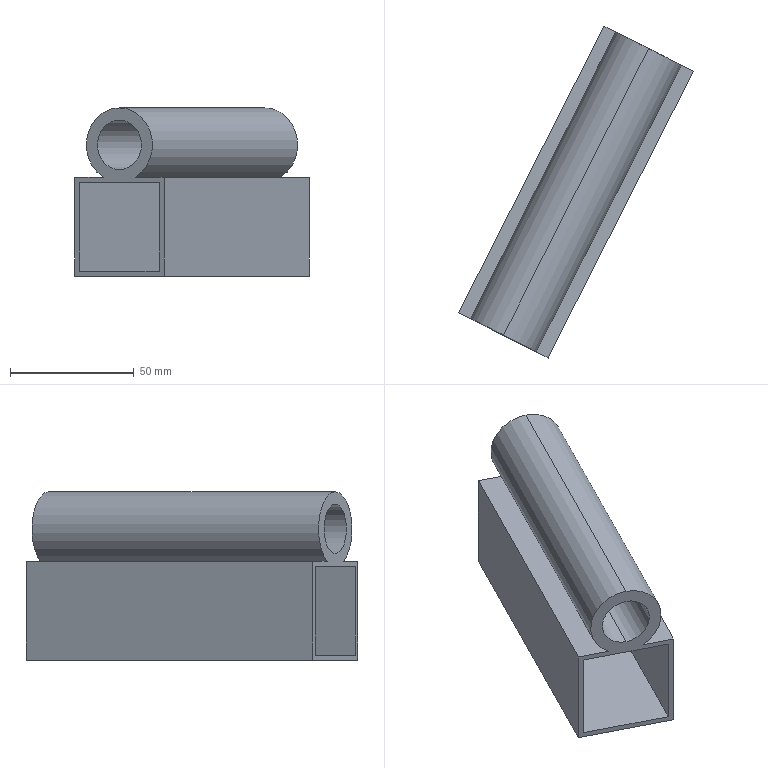Component | SolidWorks | Assembly4-1_Part24-1 | 1 solid | 15 faces | box 94.94 x 134.29 x 68.11 mm | volume 90975 mm3 | plane 11 | cylinder 4 | commonest cylinder face diameters 20 x2 30 x2
build123d program:
from build123d import *

# Parameters (mm, degrees)
SKETCH3_R           = 10
SKETCH3_W           = 36
SKETCH3_H           = 36
BOSS_EXTRUDE5_DEPTH = 130


with BuildPart() as part:
    # Sketch3 → Boss-Extrude5 (new body)
    with BuildSketch(Plane.XY):
        with BuildLine():
            Line((-59.292, 37.231), (-19.292, 37.231))
            Line((-19.292, 37.231), (-19.292, -3.313))
            Line((-19.292, -3.313), (-59.292, -3.313))
            Line((-59.292, -3.313), (-59.292, 9.667))
            ThreePointArc((-59.292, 9.667), (-87.4, 16.959), (-59.292, 24.251))
            Line((-59.292, 24.251), (-59.292, 37.231))
        make_face()
        with Locations((-72.4, 16.959)):
            Circle(SKETCH3_R, mode=Mode.SUBTRACT)
        with Locations((-39.292, 16.959)):
            Rectangle(SKETCH3_W, SKETCH3_H, mode=Mode.SUBTRACT)
    extrude(amount=BOSS_EXTRUDE5_DEPTH)


solid = part.part

# Placed as in the assembly
solid = solid.moved(Location((-428.429, -861.036, 1016.679), (90, -26.879, -90)))
STEP:
#1=CARTESIAN_POINT('',(-18.586,-38.766,43.271));
#2=VERTEX_POINT('',#1);
#3=CARTESIAN_POINT('',(-18.586,-38.766,42.483));
#4=VERTEX_POINT('',#3);
#5=CARTESIAN_POINT('',(-18.586,-38.766,42.877));
#6=DIRECTION('',(-0.4521,-0.892,-0.));
#7=DIRECTION('',(0.,0.,-1.));
#8=AXIS2_PLACEMENT_3D('',#5,#6,#7);
#9=CIRCLE('',#8,0.3937);
#10=EDGE_CURVE('',#2,#4,#9,.T.);
#11=ORIENTED_EDGE('',*,*,#10,.T.);
#12=CARTESIAN_POINT('',(-16.272,-34.201,42.483));
#13=VERTEX_POINT('',#12);
#14=CARTESIAN_POINT('',(-18.586,-38.766,42.483));
#15=DIRECTION('',(0.4521,0.892,0.));
#16=VECTOR('',#15,39.37);
#17=LINE('',#14,#16);
#18=EDGE_CURVE('',#4,#13,#17,.T.);
#19=ORIENTED_EDGE('',*,*,#18,.T.);
#20=CARTESIAN_POINT('',(-16.272,-34.201,43.271));
#21=VERTEX_POINT('',#20);
#22=CARTESIAN_POINT('',(-16.272,-34.201,42.877));
#23=DIRECTION('',(-0.4521,-0.892,-0.));
#24=DIRECTION('',(0.,0.,-1.));
#25=AXIS2_PLACEMENT_3D('',#22,#23,#24);
#26=CIRCLE('',#25,0.3937);
#27=EDGE_CURVE('',#21,#13,#26,.T.);
#28=ORIENTED_EDGE('',*,*,#27,.F.);
#29=CARTESIAN_POINT('',(-18.586,-38.766,43.271));
#30=DIRECTION('',(0.4521,0.892,0.));
#31=VECTOR('',#30,39.37);
#32=LINE('',#29,#31);
#33=EDGE_CURVE('',#2,#21,#32,.T.);
#34=ORIENTED_EDGE('',*,*,#33,.F.);
#35=EDGE_LOOP('',(#11,#19,#28,#34));
#36=FACE_OUTER_BOUND('',#35,.T.);
#37=CARTESIAN_POINT('',(-18.586,-38.766,42.877));
#38=DIRECTION('',(0.4521,0.892,0.));
#39=DIRECTION('',(-0.,-0.,1.));
#40=AXIS2_PLACEMENT_3D('',#37,#38,#39);
#41=CYLINDRICAL_SURFACE('',#40,0.3937);
#42=ADVANCED_FACE('',(#36),#41,.F.);
#43=CARTESIAN_POINT('',(-18.586,-38.766,43.468));
#44=VERTEX_POINT('',#43);
#45=CARTESIAN_POINT('',(-18.842,-38.636,42.361));
#46=VERTEX_POINT('',#45);
#47=CARTESIAN_POINT('',(-18.586,-38.766,42.877));
#48=DIRECTION('',(-0.4521,-0.892,-0.));
#49=DIRECTION('',(0.,0.,-1.));
#50=AXIS2_PLACEMENT_3D('',#47,#48,#49);
#51=CIRCLE('',#50,0.5906);
#52=EDGE_CURVE('',#44,#46,#51,.T.);
#53=ORIENTED_EDGE('',*,*,#52,.F.);
#54=CARTESIAN_POINT('',(-16.272,-34.201,43.468));
#55=VERTEX_POINT('',#54);
#56=CARTESIAN_POINT('',(-18.586,-38.766,43.468));
#57=DIRECTION('',(0.4521,0.892,0.));
#58=VECTOR('',#57,39.37);
#59=LINE('',#56,#58);
#60=EDGE_CURVE('',#44,#55,#59,.T.);
#61=ORIENTED_EDGE('',*,*,#60,.T.);
#62=CARTESIAN_POINT('',(-16.528,-34.071,42.361));
#63=VERTEX_POINT('',#62);
#64=CARTESIAN_POINT('',(-16.272,-34.201,42.877));
#65=DIRECTION('',(-0.4521,-0.892,-0.));
#66=DIRECTION('',(0.,0.,-1.));
#67=AXIS2_PLACEMENT_3D('',#64,#65,#66);
#68=CIRCLE('',#67,0.5906);
#69=EDGE_CURVE('',#55,#63,#68,.T.);
#70=ORIENTED_EDGE('',*,*,#69,.T.);
#71=CARTESIAN_POINT('',(-18.842,-38.636,42.361));
#72=DIRECTION('',(0.4521,0.892,0.));
#73=VECTOR('',#72,39.37);
#74=LINE('',#71,#73);
#75=EDGE_CURVE('',#46,#63,#74,.T.);
#76=ORIENTED_EDGE('',*,*,#75,.F.);
#77=EDGE_LOOP('',(#53,#61,#70,#76));
#78=FACE_OUTER_BOUND('',#77,.T.);
#79=CARTESIAN_POINT('',(-18.586,-38.766,42.877));
#80=DIRECTION('',(0.4521,0.892,0.));
#81=DIRECTION('',(-0.,-0.,1.));
#82=AXIS2_PLACEMENT_3D('',#79,#80,#81);
#83=CYLINDRICAL_SURFACE('',#82,0.5906);
#84=ADVANCED_FACE('',(#78),#83,.T.);
#85=CARTESIAN_POINT('',(-17.874,-39.127,42.361));
#86=VERTEX_POINT('',#85);
#87=CARTESIAN_POINT('',(-18.33,-38.896,42.361));
#88=VERTEX_POINT('',#87);
#89=CARTESIAN_POINT('',(-17.874,-39.127,42.361));
#90=DIRECTION('',(-0.892,0.4521,0.));
#91=VECTOR('',#90,39.37);
#92=LINE('',#89,#91);
#93=EDGE_CURVE('',#86,#88,#92,.T.);
#94=ORIENTED_EDGE('',*,*,#93,.T.);
#95=CARTESIAN_POINT('',(-18.586,-38.766,42.877));
#96=DIRECTION('',(-0.4521,-0.892,-0.));
#97=DIRECTION('',(0.,0.,-1.));
#98=AXIS2_PLACEMENT_3D('',#95,#96,#97);
#99=CIRCLE('',#98,0.5906);
#100=EDGE_CURVE('',#88,#44,#99,.T.);
#101=ORIENTED_EDGE('',*,*,#100,.T.);
#102=ORIENTED_EDGE('',*,*,#52,.T.);
#103=CARTESIAN_POINT('',(-19.297,-38.405,42.361));
#104=VERTEX_POINT('',#103);
#105=CARTESIAN_POINT('',(-18.842,-38.636,42.361));
#106=DIRECTION('',(-0.892,0.4521,0.));
#107=VECTOR('',#106,39.37);
#108=LINE('',#105,#107);
#109=EDGE_CURVE('',#46,#104,#108,.T.);
#110=ORIENTED_EDGE('',*,*,#109,.T.);
#111=CARTESIAN_POINT('',(-19.297,-38.405,40.786));
#112=VERTEX_POINT('',#111);
#113=CARTESIAN_POINT('',(-19.297,-38.405,42.361));
#114=DIRECTION('',(0.,0.,-1.));
#115=VECTOR('',#114,39.37);
#116=LINE('',#113,#115);
#117=EDGE_CURVE('',#104,#112,#116,.T.);
#118=ORIENTED_EDGE('',*,*,#117,.T.);
#119=CARTESIAN_POINT('',(-17.874,-39.127,40.786));
#120=VERTEX_POINT('',#119);
#121=CARTESIAN_POINT('',(-17.874,-39.127,40.786));
#122=DIRECTION('',(0.892,-0.4521,-0.));
#123=VECTOR('',#122,39.37);
#124=LINE('',#121,#123);
#125=EDGE_CURVE('',#112,#120,#124,.T.);
#126=ORIENTED_EDGE('',*,*,#125,.T.);
#127=CARTESIAN_POINT('',(-17.874,-39.127,42.361));
#128=DIRECTION('',(-0.,-0.,1.));
#129=VECTOR('',#128,39.37);
#130=LINE('',#127,#129);
#131=EDGE_CURVE('',#120,#86,#130,.T.);
#132=ORIENTED_EDGE('',*,*,#131,.T.);
#133=EDGE_LOOP('',(#94,#101,#102,#110,#118,#126,#132));
#134=FACE_OUTER_BOUND('',#133,.T.);
#135=ORIENTED_EDGE('',*,*,#10,.F.);
#136=CARTESIAN_POINT('',(-18.586,-38.766,42.877));
#137=DIRECTION('',(-0.4521,-0.892,-0.));
#138=DIRECTION('',(0.,0.,-1.));
#139=AXIS2_PLACEMENT_3D('',#136,#137,#138);
#140=CIRCLE('',#139,0.3937);
#141=EDGE_CURVE('',#4,#2,#140,.T.);
#142=ORIENTED_EDGE('',*,*,#141,.F.);
#143=EDGE_LOOP('',(#135,#142));
#144=FACE_BOUND('',#143,.T.);
#145=CARTESIAN_POINT('',(-17.954,-39.086,40.865));
#146=VERTEX_POINT('',#145);
#147=CARTESIAN_POINT('',(-17.954,-39.086,42.282));
#148=VERTEX_POINT('',#147);
#149=CARTESIAN_POINT('',(-17.954,-39.086,42.282));
#150=DIRECTION('',(-0.,-0.,1.));
#151=VECTOR('',#150,39.37);
#152=LINE('',#149,#151);
#153=EDGE_CURVE('',#146,#148,#152,.T.);
#154=ORIENTED_EDGE('',*,*,#153,.F.);
#155=CARTESIAN_POINT('',(-19.218,-38.446,40.865));
#156=VERTEX_POINT('',#155);
#157=CARTESIAN_POINT('',(-17.954,-39.086,40.865));
#158=DIRECTION('',(0.892,-0.4521,-0.));
#159=VECTOR('',#158,39.37);
#160=LINE('',#157,#159);
#161=EDGE_CURVE('',#156,#146,#160,.T.);
#162=ORIENTED_EDGE('',*,*,#161,.F.);
#163=CARTESIAN_POINT('',(-19.218,-38.446,42.282));
#164=VERTEX_POINT('',#163);
#165=CARTESIAN_POINT('',(-19.218,-38.446,42.282));
#166=DIRECTION('',(0.,0.,-1.));
#167=VECTOR('',#166,39.37);
#168=LINE('',#165,#167);
#169=EDGE_CURVE('',#164,#156,#168,.T.);
#170=ORIENTED_EDGE('',*,*,#169,.F.);
#171=CARTESIAN_POINT('',(-17.954,-39.086,42.282));
#172=DIRECTION('',(-0.892,0.4521,0.));
#173=VECTOR('',#172,39.37);
#174=LINE('',#171,#173);
#175=EDGE_CURVE('',#148,#164,#174,.T.);
#176=ORIENTED_EDGE('',*,*,#175,.F.);
#177=EDGE_LOOP('',(#154,#162,#170,#176));
#178=FACE_BOUND('',#177,.T.);
#179=CARTESIAN_POINT('',(-18.586,-38.766,42.877));
#180=DIRECTION('',(-0.4521,-0.892,-0.));
#181=DIRECTION('',(0.,0.,-1.));
#182=AXIS2_PLACEMENT_3D('',#179,#180,#181);
#183=PLANE('',#182);
#184=ADVANCED_FACE('',(#134,#144,#178),#183,.T.);
#185=ORIENTED_EDGE('',*,*,#27,.T.);
#186=CARTESIAN_POINT('',(-16.272,-34.201,42.877));
#187=DIRECTION('',(-0.4521,-0.892,-0.));
#188=DIRECTION('',(0.,0.,-1.));
#189=AXIS2_PLACEMENT_3D('',#186,#187,#188);
#190=CIRCLE('',#189,0.3937);
#191=EDGE_CURVE('',#13,#21,#190,.T.);
#192=ORIENTED_EDGE('',*,*,#191,.T.);
#193=EDGE_LOOP('',(#185,#192));
#194=FACE_BOUND('',#193,.T.);
#195=CARTESIAN_POINT('',(-15.56,-34.562,42.361));
#196=VERTEX_POINT('',#195);
#197=CARTESIAN_POINT('',(-16.016,-34.331,42.361));
#198=VERTEX_POINT('',#197);
#199=CARTESIAN_POINT('',(-15.56,-34.562,42.361));
#200=DIRECTION('',(-0.892,0.4521,0.));
#201=VECTOR('',#200,39.37);
#202=LINE('',#199,#201);
#203=EDGE_CURVE('',#196,#198,#202,.T.);
#204=ORIENTED_EDGE('',*,*,#203,.F.);
#205=CARTESIAN_POINT('',(-15.56,-34.562,40.786));
#206=VERTEX_POINT('',#205);
#207=CARTESIAN_POINT('',(-15.56,-34.562,42.361));
#208=DIRECTION('',(-0.,-0.,1.));
#209=VECTOR('',#208,39.37);
#210=LINE('',#207,#209);
#211=EDGE_CURVE('',#206,#196,#210,.T.);
#212=ORIENTED_EDGE('',*,*,#211,.F.);
#213=CARTESIAN_POINT('',(-16.984,-33.84,40.786));
#214=VERTEX_POINT('',#213);
#215=CARTESIAN_POINT('',(-15.56,-34.562,40.786));
#216=DIRECTION('',(0.892,-0.4521,-0.));
#217=VECTOR('',#216,39.37);
#218=LINE('',#215,#217);
#219=EDGE_CURVE('',#214,#206,#218,.T.);
#220=ORIENTED_EDGE('',*,*,#219,.F.);
#221=CARTESIAN_POINT('',(-16.984,-33.84,42.361));
#222=VERTEX_POINT('',#221);
#223=CARTESIAN_POINT('',(-16.984,-33.84,42.361));
#224=DIRECTION('',(0.,0.,-1.));
#225=VECTOR('',#224,39.37);
#226=LINE('',#223,#225);
#227=EDGE_CURVE('',#222,#214,#226,.T.);
#228=ORIENTED_EDGE('',*,*,#227,.F.);
#229=CARTESIAN_POINT('',(-16.528,-34.071,42.361));
#230=DIRECTION('',(-0.892,0.4521,0.));
#231=VECTOR('',#230,39.37);
#232=LINE('',#229,#231);
#233=EDGE_CURVE('',#63,#222,#232,.T.);
#234=ORIENTED_EDGE('',*,*,#233,.F.);
#235=ORIENTED_EDGE('',*,*,#69,.F.);
#236=CARTESIAN_POINT('',(-16.272,-34.201,42.877));
#237=DIRECTION('',(-0.4521,-0.892,-0.));
#238=DIRECTION('',(0.,0.,-1.));
#239=AXIS2_PLACEMENT_3D('',#236,#237,#238);
#240=CIRCLE('',#239,0.5906);
#241=EDGE_CURVE('',#198,#55,#240,.T.);
#242=ORIENTED_EDGE('',*,*,#241,.F.);
#243=EDGE_LOOP('',(#204,#212,#220,#228,#234,#235,#242));
#244=FACE_OUTER_BOUND('',#243,.T.);
#245=CARTESIAN_POINT('',(-16.904,-33.881,40.865));
#246=VERTEX_POINT('',#245);
#247=CARTESIAN_POINT('',(-15.64,-34.521,40.865));
#248=VERTEX_POINT('',#247);
#249=CARTESIAN_POINT('',(-15.64,-34.521,40.865));
#250=DIRECTION('',(0.892,-0.4521,-0.));
#251=VECTOR('',#250,39.37);
#252=LINE('',#249,#251);
#253=EDGE_CURVE('',#246,#248,#252,.T.);
#254=ORIENTED_EDGE('',*,*,#253,.T.);
#255=CARTESIAN_POINT('',(-15.64,-34.521,42.282));
#256=VERTEX_POINT('',#255);
#257=CARTESIAN_POINT('',(-15.64,-34.521,42.282));
#258=DIRECTION('',(-0.,-0.,1.));
#259=VECTOR('',#258,39.37);
#260=LINE('',#257,#259);
#261=EDGE_CURVE('',#248,#256,#260,.T.);
#262=ORIENTED_EDGE('',*,*,#261,.T.);
#263=CARTESIAN_POINT('',(-16.904,-33.881,42.282));
#264=VERTEX_POINT('',#263);
#265=CARTESIAN_POINT('',(-15.64,-34.521,42.282));
#266=DIRECTION('',(-0.892,0.4521,0.));
#267=VECTOR('',#266,39.37);
#268=LINE('',#265,#267);
#269=EDGE_CURVE('',#256,#264,#268,.T.);
#270=ORIENTED_EDGE('',*,*,#269,.T.);
#271=CARTESIAN_POINT('',(-16.904,-33.881,42.282));
#272=DIRECTION('',(0.,0.,-1.));
#273=VECTOR('',#272,39.37);
#274=LINE('',#271,#273);
#275=EDGE_CURVE('',#264,#246,#274,.T.);
#276=ORIENTED_EDGE('',*,*,#275,.T.);
#277=EDGE_LOOP('',(#254,#262,#270,#276));
#278=FACE_BOUND('',#277,.T.);
#279=CARTESIAN_POINT('',(-16.272,-34.201,42.877));
#280=DIRECTION('',(-0.4521,-0.892,-0.));
#281=DIRECTION('',(0.,0.,-1.));
#282=AXIS2_PLACEMENT_3D('',#279,#280,#281);
#283=PLANE('',#282);
#284=ADVANCED_FACE('',(#194,#244,#278),#283,.F.);
#285=ORIENTED_EDGE('',*,*,#203,.T.);
#286=CARTESIAN_POINT('',(-18.33,-38.896,42.361));
#287=DIRECTION('',(0.4521,0.892,0.));
#288=VECTOR('',#287,39.37);
#289=LINE('',#286,#288);
#290=EDGE_CURVE('',#88,#198,#289,.T.);
#291=ORIENTED_EDGE('',*,*,#290,.F.);
#292=ORIENTED_EDGE('',*,*,#93,.F.);
#293=CARTESIAN_POINT('',(-17.874,-39.127,42.361));
#294=DIRECTION('',(0.4521,0.892,0.));
#295=VECTOR('',#294,39.37);
#296=LINE('',#293,#295);
#297=EDGE_CURVE('',#86,#196,#296,.T.);
#298=ORIENTED_EDGE('',*,*,#297,.T.);
#299=EDGE_LOOP('',(#285,#291,#292,#298));
#300=FACE_OUTER_BOUND('',#299,.T.);
#301=CARTESIAN_POINT('',(-17.874,-39.127,42.361));
#302=DIRECTION('',(0.,0.,-1.));
#303=DIRECTION('',(0.892,-0.4521,-0.));
#304=AXIS2_PLACEMENT_3D('',#301,#302,#303);
#305=PLANE('',#304);
#306=ADVANCED_FACE('',(#300),#305,.F.);
#307=ORIENTED_EDGE('',*,*,#60,.F.);
#308=ORIENTED_EDGE('',*,*,#100,.F.);
#309=ORIENTED_EDGE('',*,*,#290,.T.);
#310=ORIENTED_EDGE('',*,*,#241,.T.);
#311=EDGE_LOOP('',(#307,#308,#309,#310));
#312=FACE_OUTER_BOUND('',#311,.T.);
#313=CARTESIAN_POINT('',(-18.586,-38.766,42.877));
#314=DIRECTION('',(0.4521,0.892,0.));
#315=DIRECTION('',(-0.,-0.,1.));
#316=AXIS2_PLACEMENT_3D('',#313,#314,#315);
#317=CYLINDRICAL_SURFACE('',#316,0.5906);
#318=ADVANCED_FACE('',(#312),#317,.T.);
#319=ORIENTED_EDGE('',*,*,#233,.T.);
#320=CARTESIAN_POINT('',(-19.297,-38.405,42.361));
#321=DIRECTION('',(0.4521,0.892,0.));
#322=VECTOR('',#321,39.37);
#323=LINE('',#320,#322);
#324=EDGE_CURVE('',#104,#222,#323,.T.);
#325=ORIENTED_EDGE('',*,*,#324,.F.);
#326=ORIENTED_EDGE('',*,*,#109,.F.);
#327=ORIENTED_EDGE('',*,*,#75,.T.);
#328=EDGE_LOOP('',(#319,#325,#326,#327));
#329=FACE_OUTER_BOUND('',#328,.T.);
#330=CARTESIAN_POINT('',(-18.842,-38.636,42.361));
#331=DIRECTION('',(0.,0.,-1.));
#332=DIRECTION('',(0.4521,0.892,0.));
#333=AXIS2_PLACEMENT_3D('',#330,#331,#332);
#334=PLANE('',#333);
#335=ADVANCED_FACE('',(#329),#334,.F.);
#336=ORIENTED_EDGE('',*,*,#227,.T.);
#337=CARTESIAN_POINT('',(-19.297,-38.405,40.786));
#338=DIRECTION('',(0.4521,0.892,0.));
#339=VECTOR('',#338,39.37);
#340=LINE('',#337,#339);
#341=EDGE_CURVE('',#112,#214,#340,.T.);
#342=ORIENTED_EDGE('',*,*,#341,.F.);
#343=ORIENTED_EDGE('',*,*,#117,.F.);
#344=ORIENTED_EDGE('',*,*,#324,.T.);
#345=EDGE_LOOP('',(#336,#342,#343,#344));
#346=FACE_OUTER_BOUND('',#345,.T.);
#347=CARTESIAN_POINT('',(-19.297,-38.405,42.361));
#348=DIRECTION('',(0.892,-0.4521,-0.));
#349=DIRECTION('',(-0.4521,-0.892,-0.));
#350=AXIS2_PLACEMENT_3D('',#347,#348,#349);
#351=PLANE('',#350);
#352=ADVANCED_FACE('',(#346),#351,.F.);
#353=ORIENTED_EDGE('',*,*,#219,.T.);
#354=CARTESIAN_POINT('',(-17.874,-39.127,40.786));
#355=DIRECTION('',(0.4521,0.892,0.));
#356=VECTOR('',#355,39.37);
#357=LINE('',#354,#356);
#358=EDGE_CURVE('',#120,#206,#357,.T.);
#359=ORIENTED_EDGE('',*,*,#358,.F.);
#360=ORIENTED_EDGE('',*,*,#125,.F.);
#361=ORIENTED_EDGE('',*,*,#341,.T.);
#362=EDGE_LOOP('',(#353,#359,#360,#361));
#363=FACE_OUTER_BOUND('',#362,.T.);
#364=CARTESIAN_POINT('',(-17.874,-39.127,40.786));
#365=DIRECTION('',(-0.,-0.,1.));
#366=DIRECTION('',(-0.892,0.4521,0.));
#367=AXIS2_PLACEMENT_3D('',#364,#365,#366);
#368=PLANE('',#367);
#369=ADVANCED_FACE('',(#363),#368,.F.);
#370=ORIENTED_EDGE('',*,*,#211,.T.);
#371=ORIENTED_EDGE('',*,*,#297,.F.);
#372=ORIENTED_EDGE('',*,*,#131,.F.);
#373=ORIENTED_EDGE('',*,*,#358,.T.);
#374=EDGE_LOOP('',(#370,#371,#372,#373));
#375=FACE_OUTER_BOUND('',#374,.T.);
#376=CARTESIAN_POINT('',(-17.874,-39.127,42.361));
#377=DIRECTION('',(-0.892,0.4521,0.));
#378=DIRECTION('',(0.,0.,-1.));
#379=AXIS2_PLACEMENT_3D('',#376,#377,#378);
#380=PLANE('',#379);
#381=ADVANCED_FACE('',(#375),#380,.F.);
#382=ORIENTED_EDGE('',*,*,#18,.F.);
#383=ORIENTED_EDGE('',*,*,#141,.T.);
#384=ORIENTED_EDGE('',*,*,#33,.T.);
#385=ORIENTED_EDGE('',*,*,#191,.F.);
#386=EDGE_LOOP('',(#382,#383,#384,#385));
#387=FACE_OUTER_BOUND('',#386,.T.);
#388=CARTESIAN_POINT('',(-18.586,-38.766,42.877));
#389=DIRECTION('',(0.4521,0.892,0.));
#390=DIRECTION('',(-0.,-0.,1.));
#391=AXIS2_PLACEMENT_3D('',#388,#389,#390);
#392=CYLINDRICAL_SURFACE('',#391,0.3937);
#393=ADVANCED_FACE('',(#387),#392,.F.);
#394=ORIENTED_EDGE('',*,*,#253,.F.);
#395=CARTESIAN_POINT('',(-19.218,-38.446,40.865));
#396=DIRECTION('',(0.4521,0.892,0.));
#397=VECTOR('',#396,39.37);
#398=LINE('',#395,#397);
#399=EDGE_CURVE('',#156,#246,#398,.T.);
#400=ORIENTED_EDGE('',*,*,#399,.F.);
#401=ORIENTED_EDGE('',*,*,#161,.T.);
#402=CARTESIAN_POINT('',(-17.954,-39.086,40.865));
#403=DIRECTION('',(0.4521,0.892,0.));
#404=VECTOR('',#403,39.37);
#405=LINE('',#402,#404);
#406=EDGE_CURVE('',#146,#248,#405,.T.);
#407=ORIENTED_EDGE('',*,*,#406,.T.);
#408=EDGE_LOOP('',(#394,#400,#401,#407));
#409=FACE_OUTER_BOUND('',#408,.T.);
#410=CARTESIAN_POINT('',(-17.954,-39.086,40.865));
#411=DIRECTION('',(-0.,-0.,1.));
#412=DIRECTION('',(-0.4521,-0.892,-0.));
#413=AXIS2_PLACEMENT_3D('',#410,#411,#412);
#414=PLANE('',#413);
#415=ADVANCED_FACE('',(#409),#414,.T.);
#416=ORIENTED_EDGE('',*,*,#261,.F.);
#417=ORIENTED_EDGE('',*,*,#406,.F.);
#418=ORIENTED_EDGE('',*,*,#153,.T.);
#419=CARTESIAN_POINT('',(-17.954,-39.086,42.282));
#420=DIRECTION('',(0.4521,0.892,0.));
#421=VECTOR('',#420,39.37);
#422=LINE('',#419,#421);
#423=EDGE_CURVE('',#148,#256,#422,.T.);
#424=ORIENTED_EDGE('',*,*,#423,.T.);
#425=EDGE_LOOP('',(#416,#417,#418,#424));
#426=FACE_OUTER_BOUND('',#425,.T.);
#427=CARTESIAN_POINT('',(-17.954,-39.086,42.282));
#428=DIRECTION('',(-0.892,0.4521,0.));
#429=DIRECTION('',(0.4521,0.892,0.));
#430=AXIS2_PLACEMENT_3D('',#427,#428,#429);
#431=PLANE('',#430);
#432=ADVANCED_FACE('',(#426),#431,.T.);
#433=ORIENTED_EDGE('',*,*,#269,.F.);
#434=ORIENTED_EDGE('',*,*,#423,.F.);
#435=ORIENTED_EDGE('',*,*,#175,.T.);
#436=CARTESIAN_POINT('',(-19.218,-38.446,42.282));
#437=DIRECTION('',(0.4521,0.892,0.));
#438=VECTOR('',#437,39.37);
#439=LINE('',#436,#438);
#440=EDGE_CURVE('',#164,#264,#439,.T.);
#441=ORIENTED_EDGE('',*,*,#440,.T.);
#442=EDGE_LOOP('',(#433,#434,#435,#441));
#443=FACE_OUTER_BOUND('',#442,.T.);
#444=CARTESIAN_POINT('',(-17.954,-39.086,42.282));
#445=DIRECTION('',(0.,0.,-1.));
#446=DIRECTION('',(0.892,-0.4521,-0.));
#447=AXIS2_PLACEMENT_3D('',#444,#445,#446);
#448=PLANE('',#447);
#449=ADVANCED_FACE('',(#443),#448,.T.);
#450=ORIENTED_EDGE('',*,*,#275,.F.);
#451=ORIENTED_EDGE('',*,*,#440,.F.);
#452=ORIENTED_EDGE('',*,*,#169,.T.);
#453=ORIENTED_EDGE('',*,*,#399,.T.);
#454=EDGE_LOOP('',(#450,#451,#452,#453));
#455=FACE_OUTER_BOUND('',#454,.T.);
#456=CARTESIAN_POINT('',(-19.218,-38.446,42.282));
#457=DIRECTION('',(0.892,-0.4521,-0.));
#458=DIRECTION('',(-0.4521,-0.892,-0.));
#459=AXIS2_PLACEMENT_3D('',#456,#457,#458);
#460=PLANE('',#459);
#461=ADVANCED_FACE('',(#455),#460,.T.);
#462=CLOSED_SHELL('',(#42,#84,#184,#284,#306,#318,#335,#352,#369,#381,#393,#415,#432,#449,#461));
#463=MANIFOLD_SOLID_BREP('',#462);
#464=CARTESIAN_POINT('',(0.,0.,0.));
#465=DIRECTION('',(0.,0.,1.));
#466=DIRECTION('',(1.,0.,0.));
#467=AXIS2_PLACEMENT_3D('',#464,#465,#466);
#468=(LENGTH_UNIT()NAMED_UNIT(*)SI_UNIT($,.METRE.));
#469=LENGTH_MEASURE_WITH_UNIT(LENGTH_MEASURE(0.0254),#468);
#470=DIMENSIONAL_EXPONENTS(1.,0.,0.,0.,0.,0.,0.);
#471=(CONVERSION_BASED_UNIT('',#469)LENGTH_UNIT()NAMED_UNIT(#470));
#472=UNCERTAINTY_MEASURE_WITH_UNIT(LENGTH_MEASURE(0.00001),#471,'','');
#473=(NAMED_UNIT(*)PLANE_ANGLE_UNIT()SI_UNIT($,.RADIAN.));
#474=(NAMED_UNIT(*)SI_UNIT($,.STERADIAN.)SOLID_ANGLE_UNIT());
#475=(GEOMETRIC_REPRESENTATION_CONTEXT(3)GLOBAL_UNCERTAINTY_ASSIGNED_CONTEXT((#472))GLOBAL_UNIT_ASSIGNED_CONTEXT((#471,#473,#474))REPRESENTATION_CONTEXT('',''));
#476=ADVANCED_BREP_SHAPE_REPRESENTATION('',(#463,#467),#475);
#477=COLOUR_RGB('',0.7922,0.8196,0.9333);
#478=FILL_AREA_STYLE_COLOUR('',#477);
#479=FILL_AREA_STYLE('',(#478));
#480=SURFACE_STYLE_FILL_AREA(#479);
#481=SURFACE_SIDE_STYLE('',(#480));
#482=SURFACE_STYLE_USAGE(.BOTH.,#481);
#483=PRESENTATION_STYLE_ASSIGNMENT((#482));
#484=STYLED_ITEM('',(#483),#463);
#485=(LENGTH_UNIT()NAMED_UNIT(*)SI_UNIT($,.METRE.));
#486=LENGTH_MEASURE_WITH_UNIT(LENGTH_MEASURE(0.0254),#485);
#487=DIMENSIONAL_EXPONENTS(1.,0.,0.,0.,0.,0.,0.);
#488=(CONVERSION_BASED_UNIT('',#486)LENGTH_UNIT()NAMED_UNIT(#487));
#489=UNCERTAINTY_MEASURE_WITH_UNIT(LENGTH_MEASURE(0.00001),#488,'','');
#490=(NAMED_UNIT(*)PLANE_ANGLE_UNIT()SI_UNIT($,.RADIAN.));
#491=(NAMED_UNIT(*)SI_UNIT($,.STERADIAN.)SOLID_ANGLE_UNIT());
#492=(GEOMETRIC_REPRESENTATION_CONTEXT(3)GLOBAL_UNCERTAINTY_ASSIGNED_CONTEXT((#489))GLOBAL_UNIT_ASSIGNED_CONTEXT((#488,#490,#491))REPRESENTATION_CONTEXT('',''));
#493=MECHANICAL_DESIGN_GEOMETRIC_PRESENTATION_REPRESENTATION('',(#484),#492);
#494=PRESENTATION_LAYER_ASSIGNMENT('','',(#484));